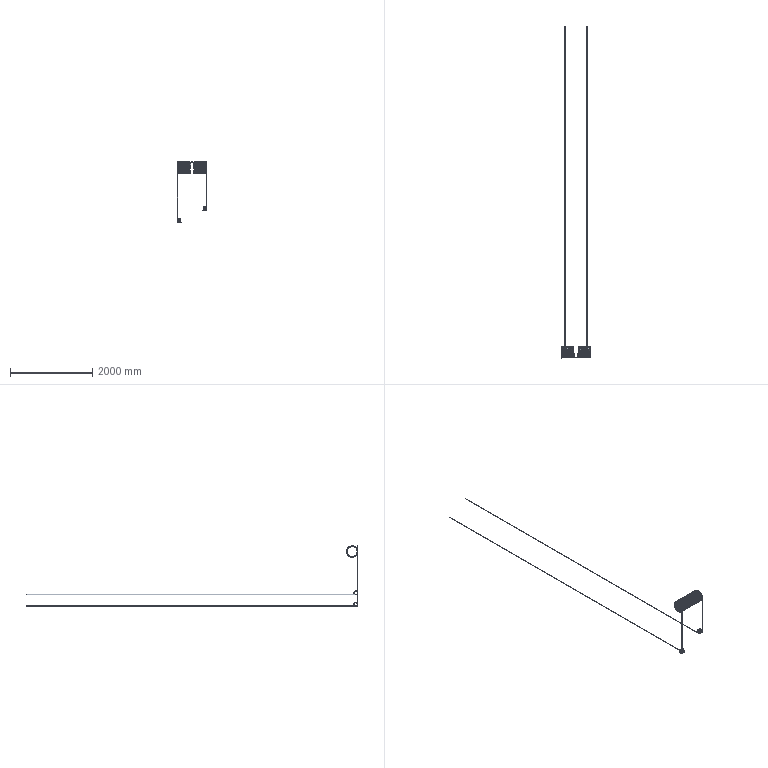Component | SolidWorks | LiftingAndOperatingMechanism-1_27-1 | 2 solids | 34 faces | volume 4359471 mm3 | plane 14 | spline 12 | cylinder 8 | commonest cylinder face diameters 10 x8